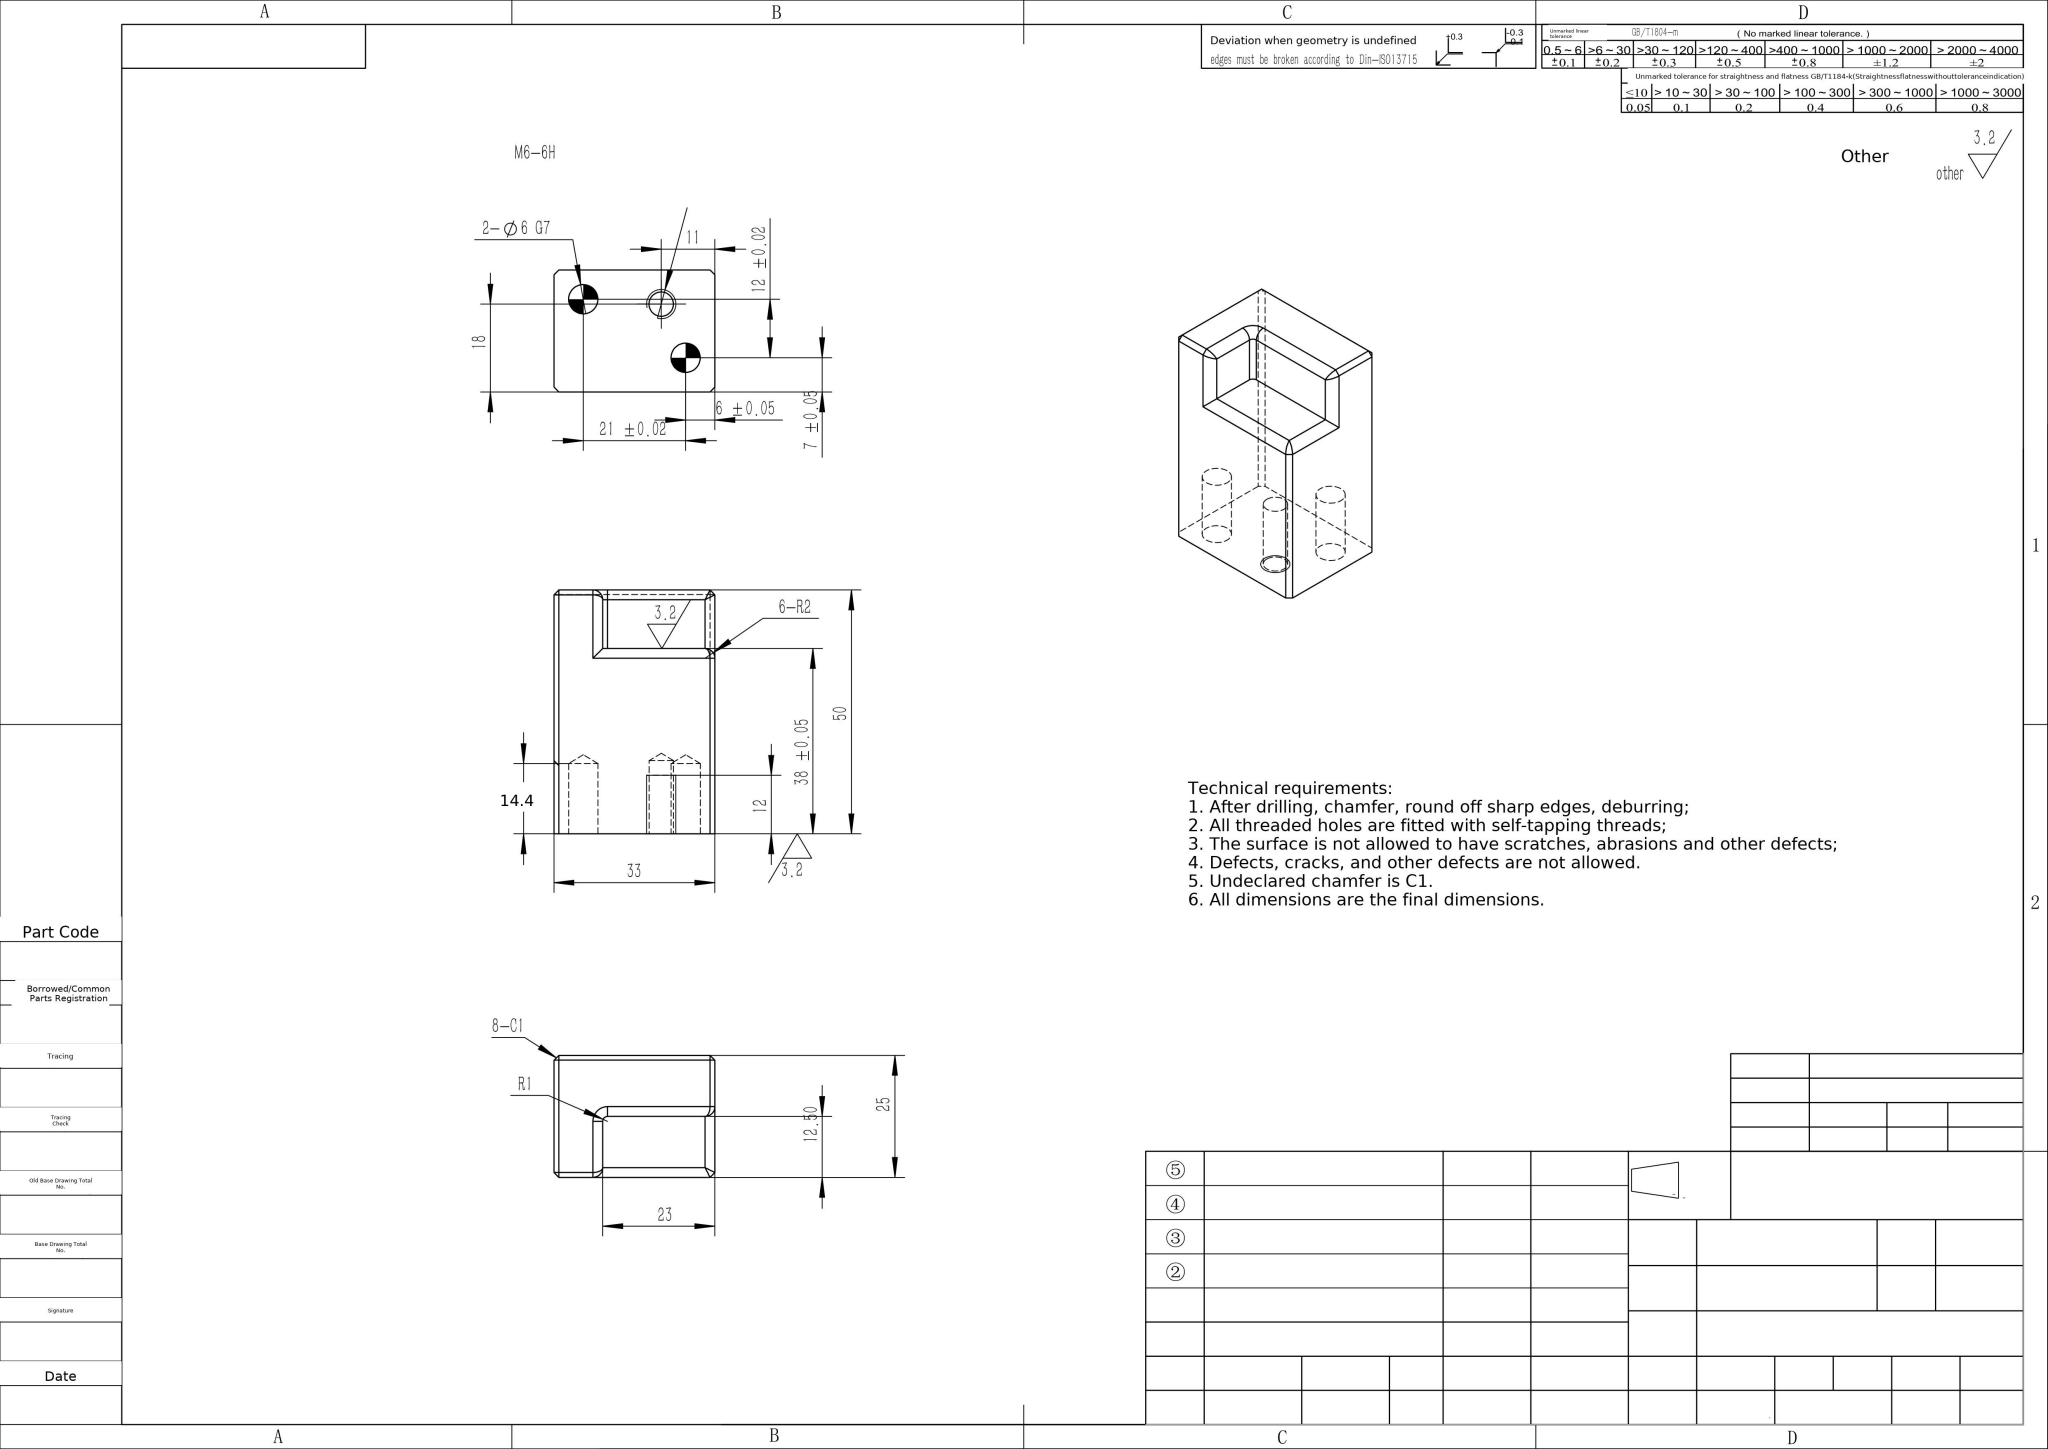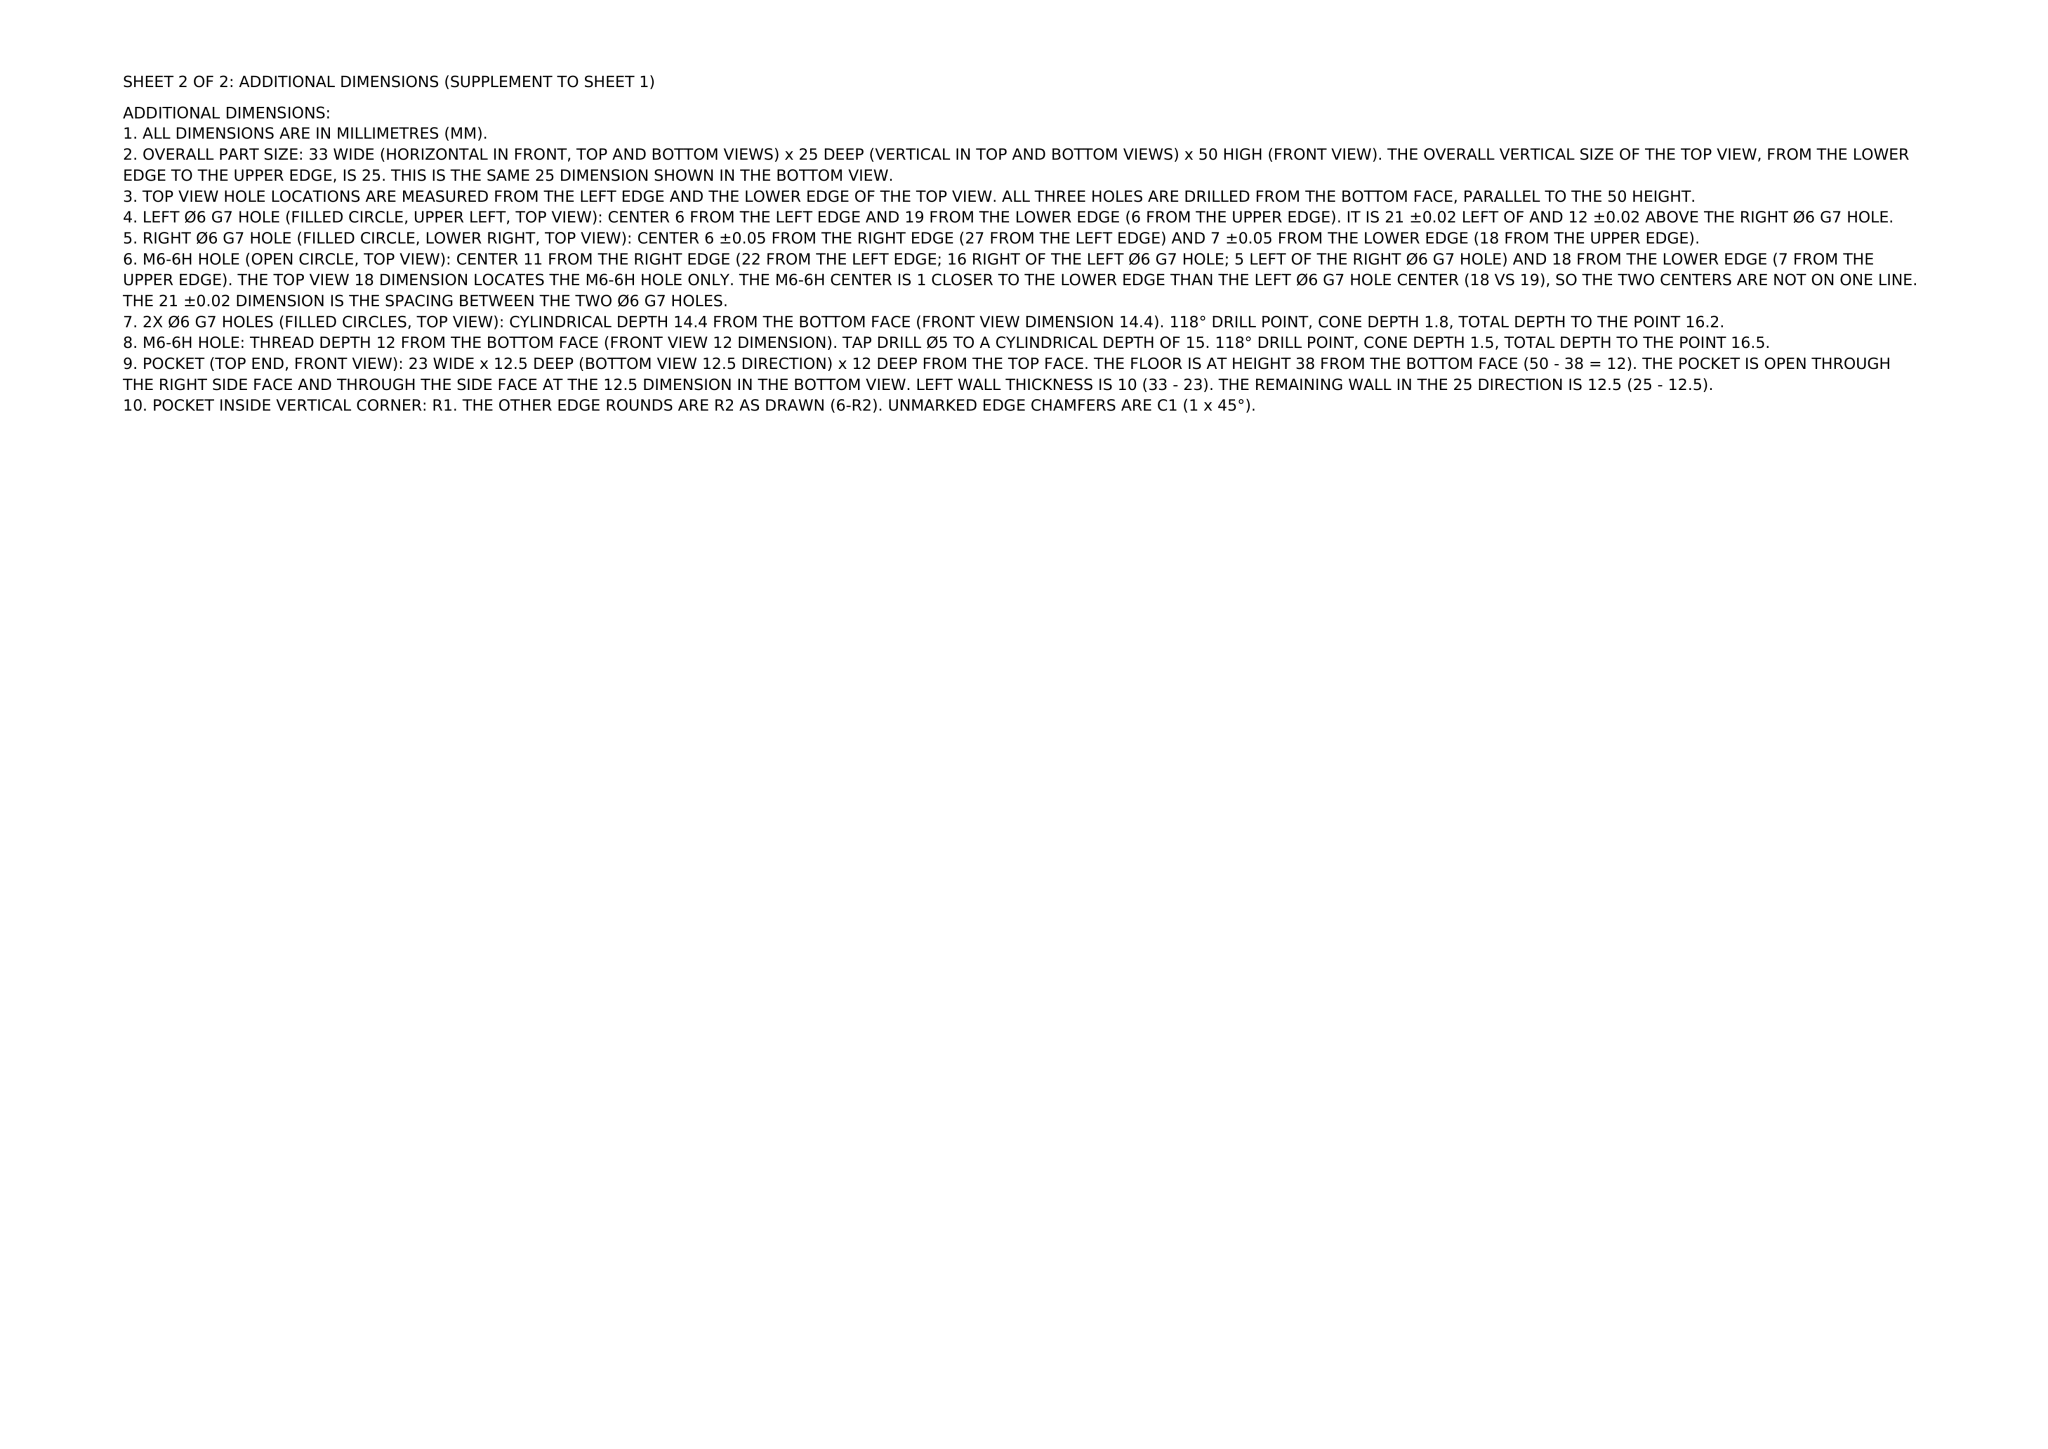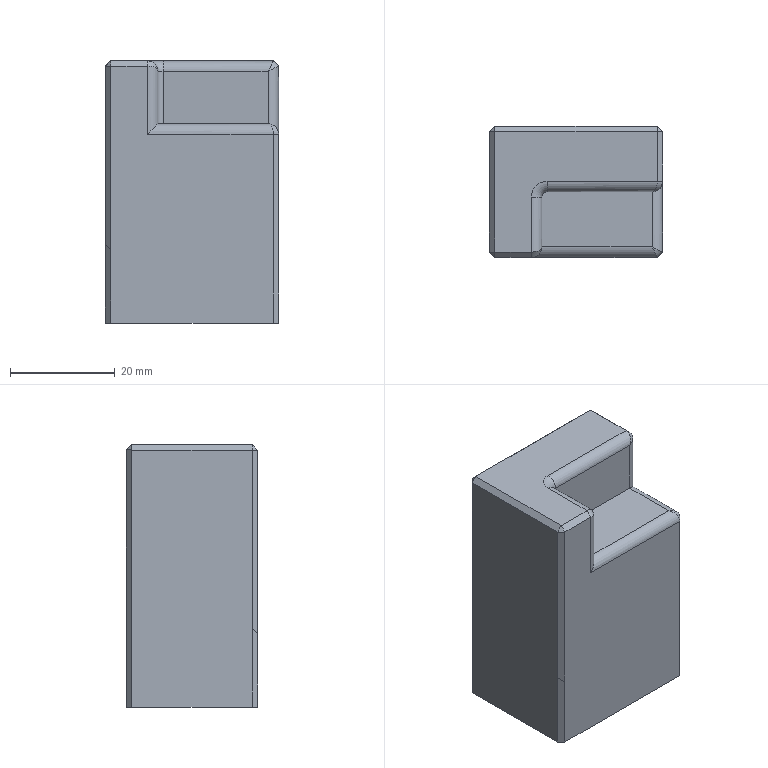Part | NX | mm | 1 solid | 44 faces | box 33 x 25 x 50 mm | volume 36444 mm3 | plane 21 | cylinder 13 | cone 6 | spline 3 | torus 1 | commonest cylinder face diameters 4 x6 6 x4 5 x2 2 x1